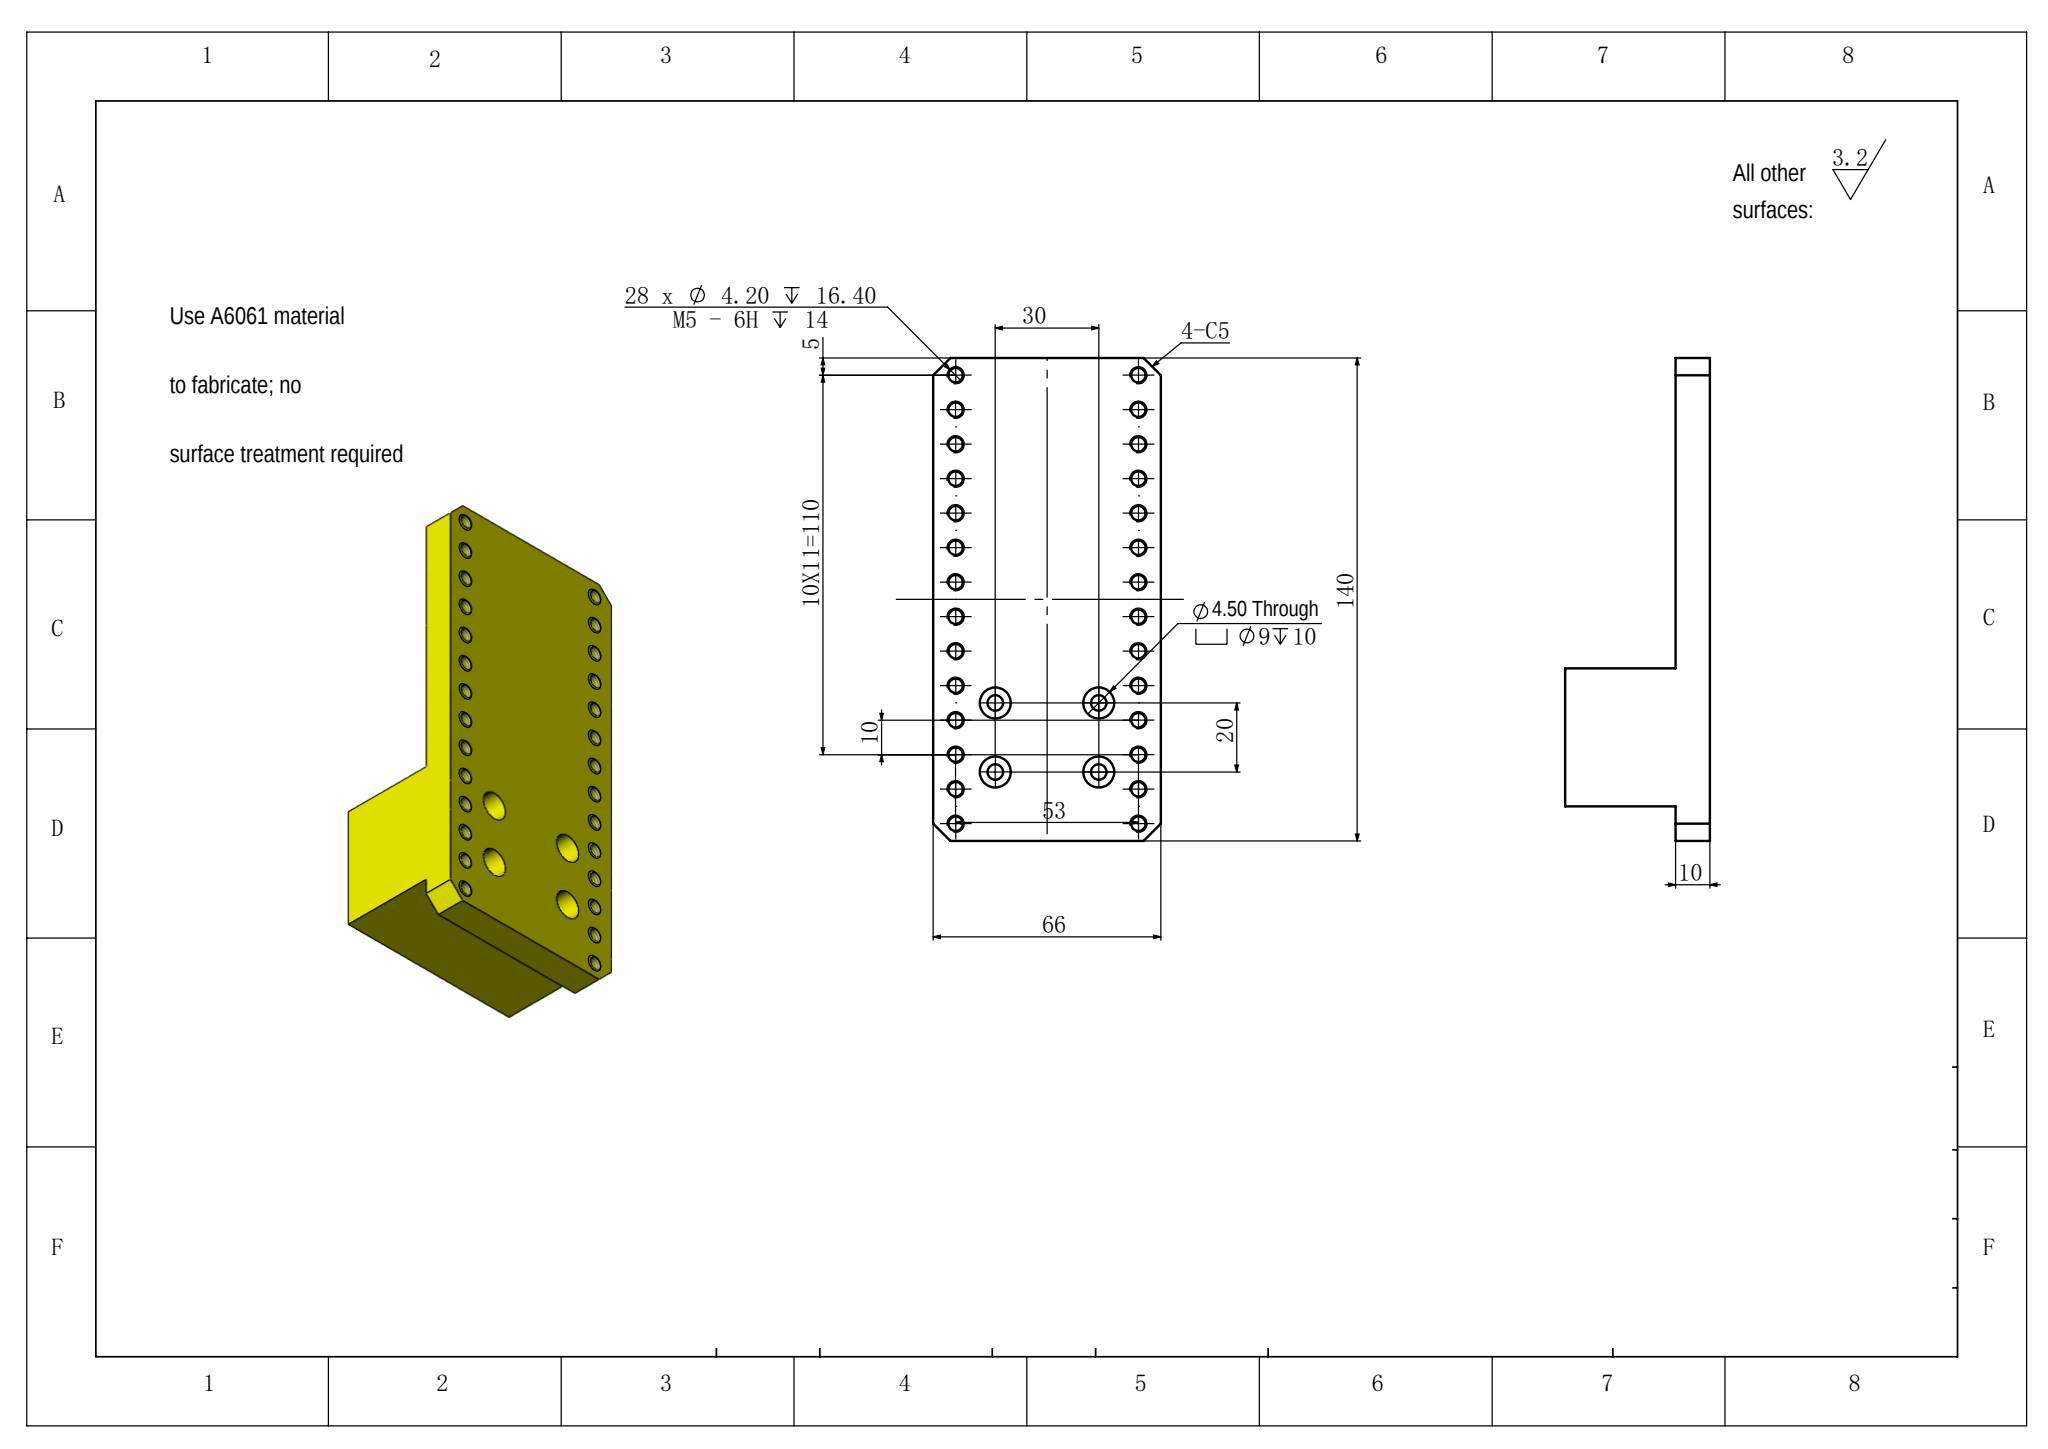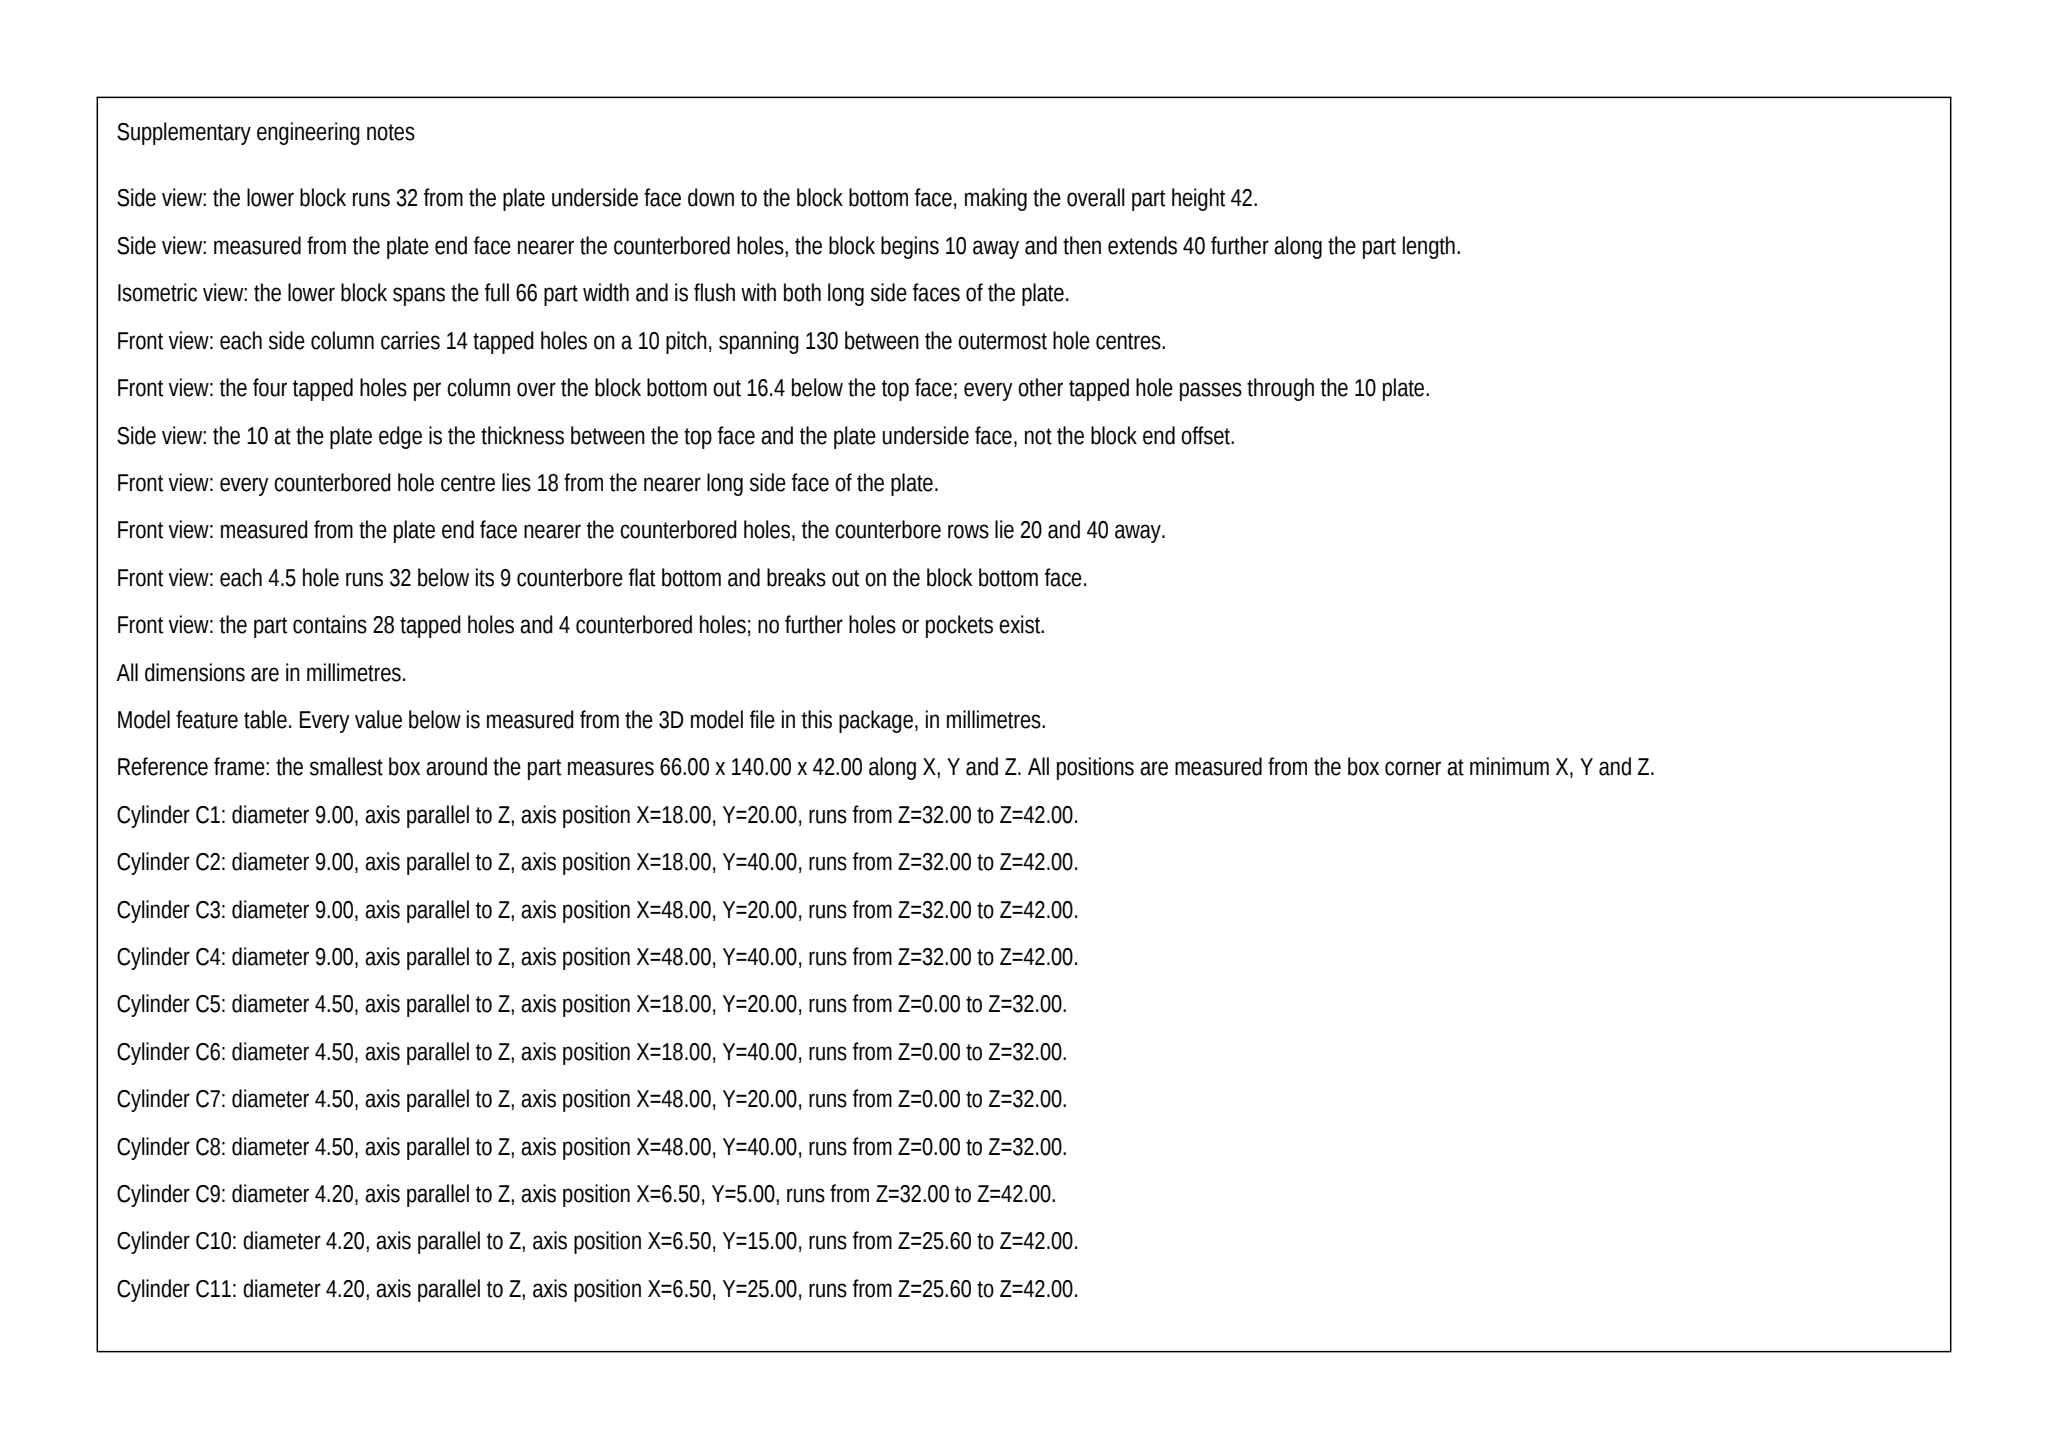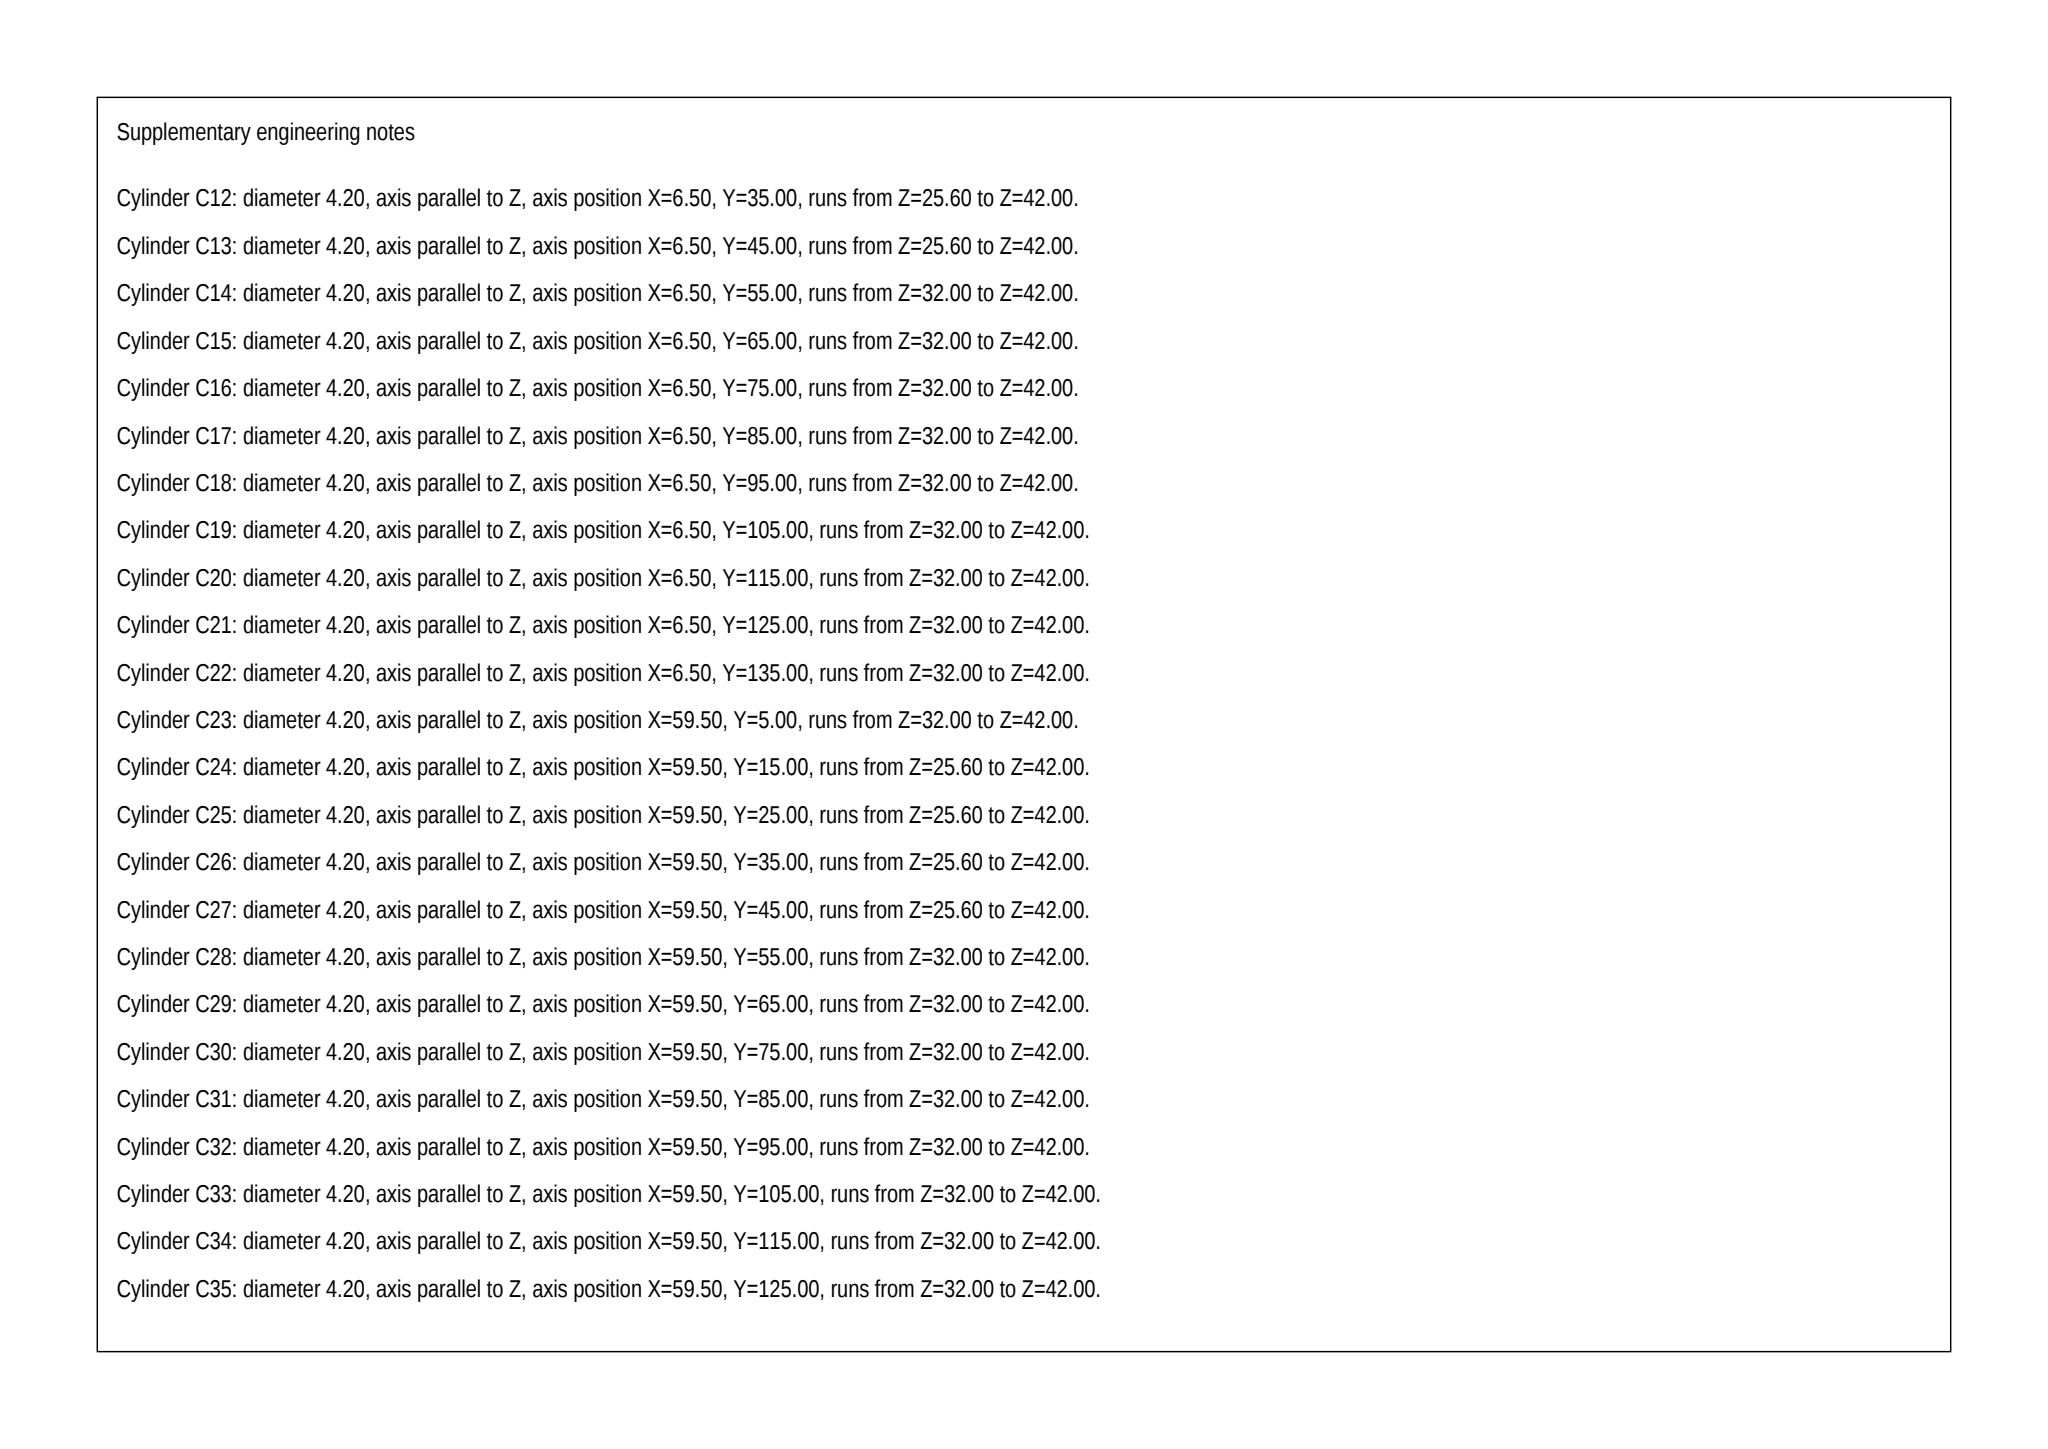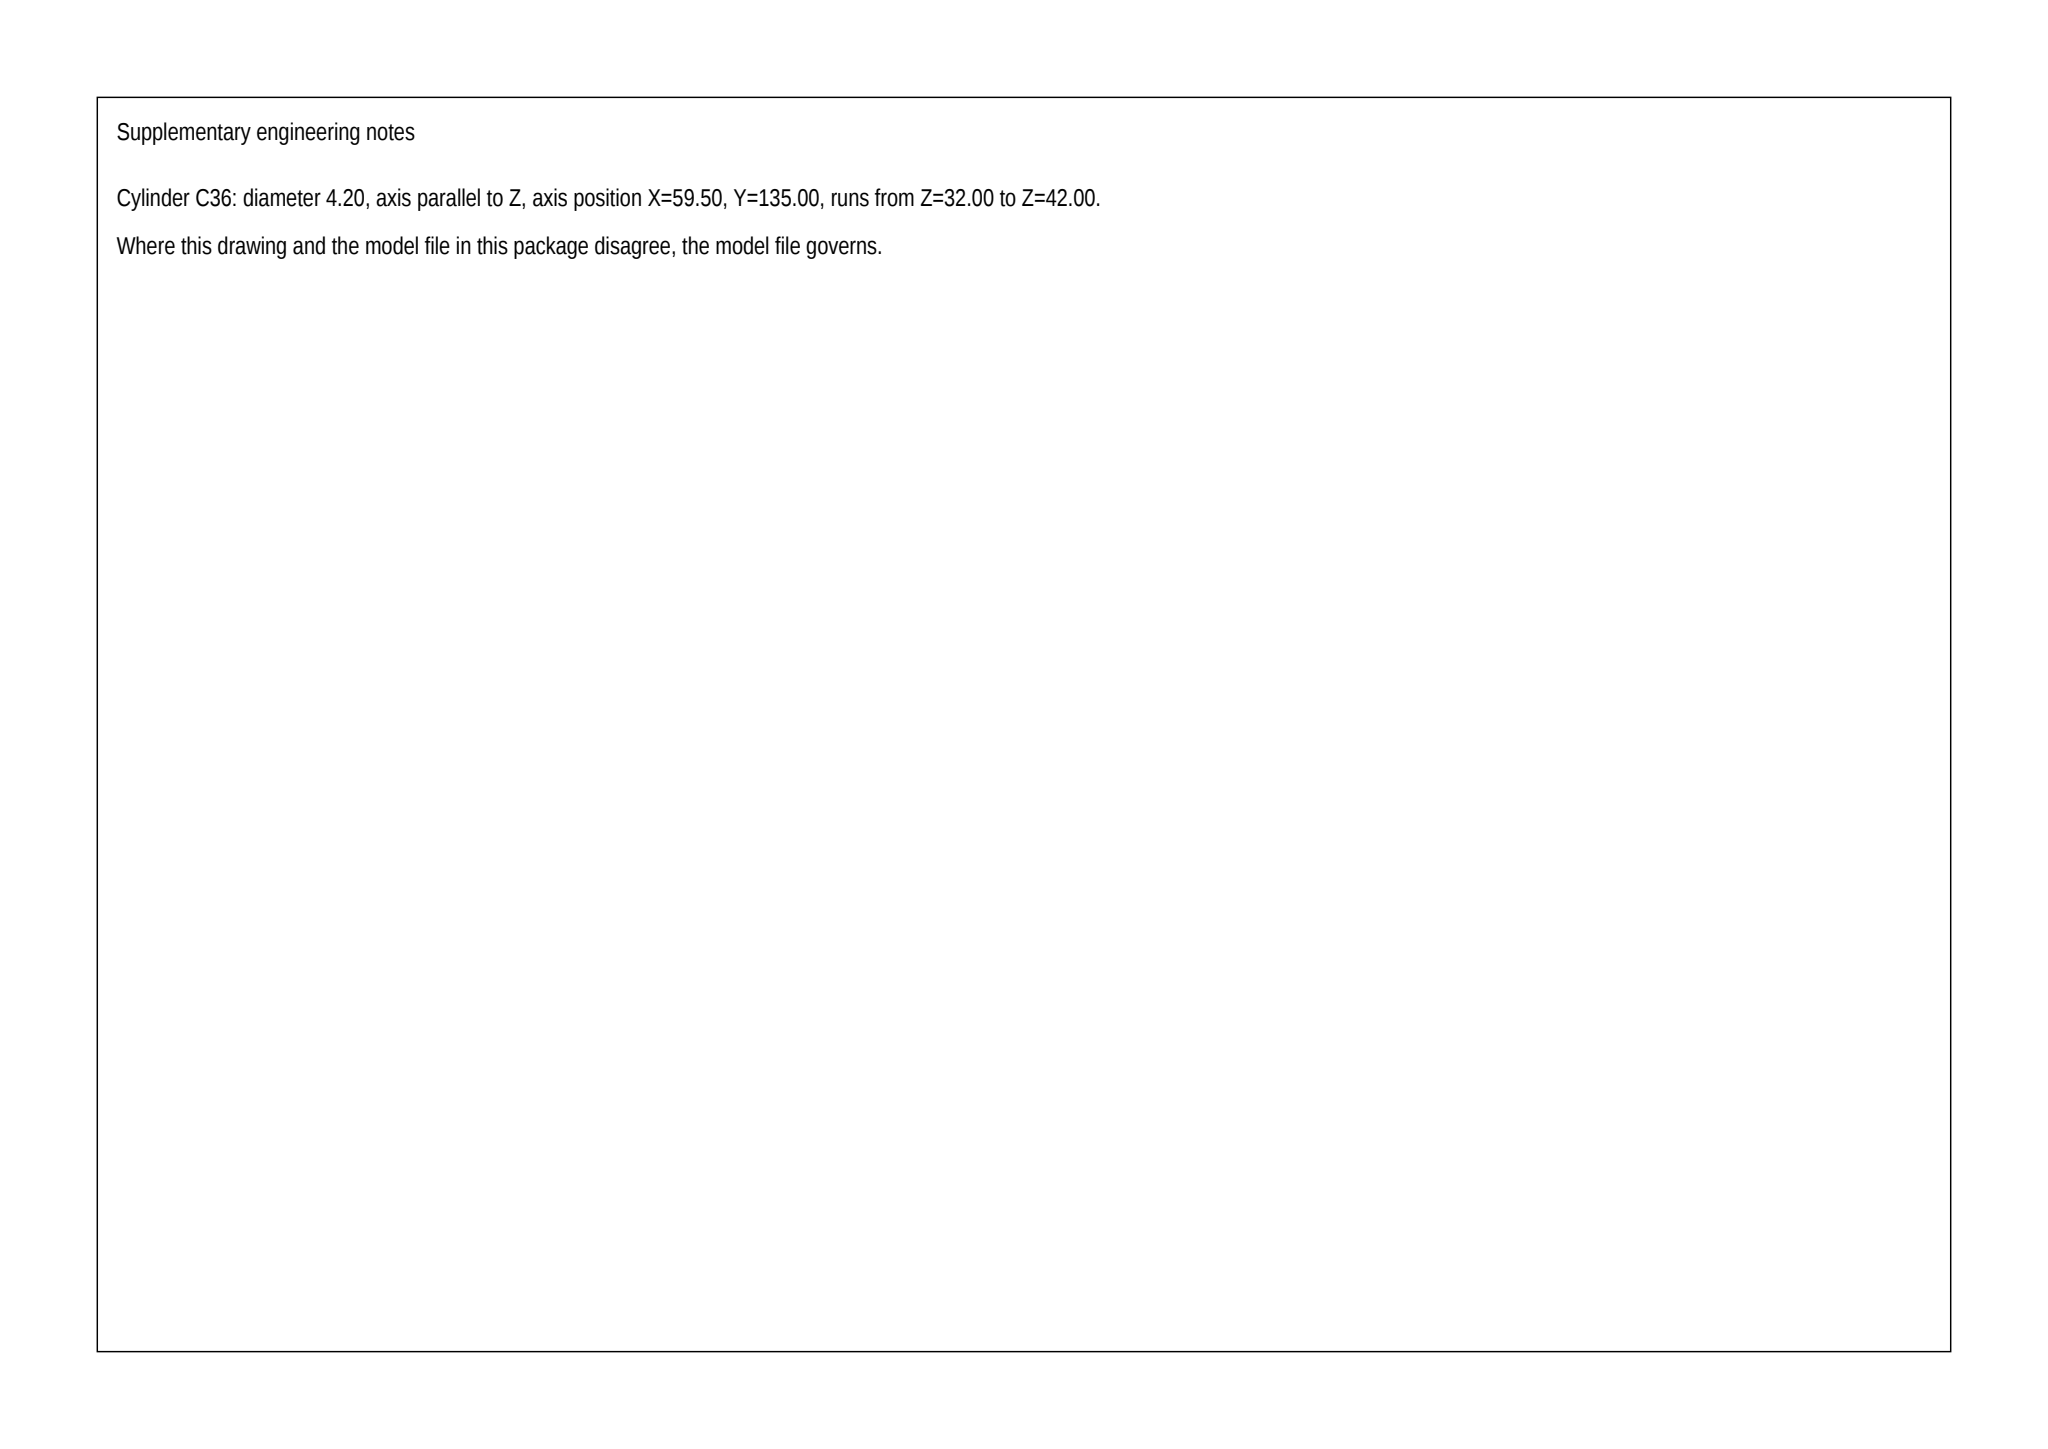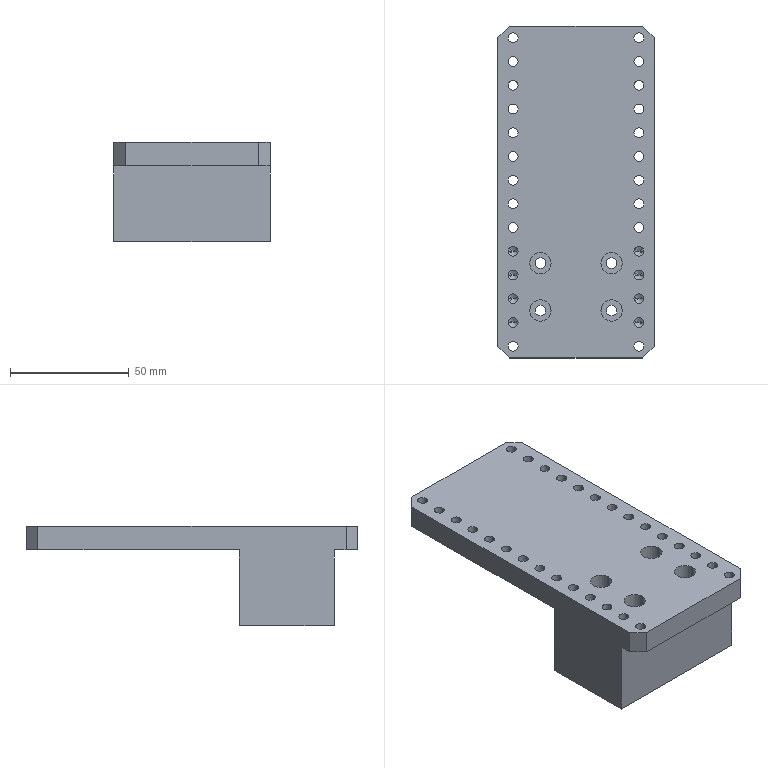Part | SolidWorks | mm | 1 solid | 106 faces | box 66 x 140 x 42 mm | volume 167164 mm3 | cylinder 72 | plane 18 | cone 16 | commonest cylinder face diameters 4.2 x56 9 x8 4.5 x8
Drawing notes:
SIDE VIEW: OVERALL DEPTH 42 | from the solid: bbox_xyz z = 42.0
BOSS PROJECTS 32 FROM PLATE BACK FACE | from the solid: z planes at 0.0 and 32.0; plate 32.0-42.0
BOSS 40 LG IN 140 DIR | from the solid: y planes at 10.0 and 50.0
BOSS STARTS 10 FROM BOTTOM EDGE | from the solid: y plane at 10.0 vs y=0 bottom edge
4X CBORED HOLES: LOWER ROW 20 FROM BOTTOM EDGE | from the solid: Ø4.5/Ø9 holes at y=20.0 and y=40.0
Ø4.50 DP 32 THRU BOSS, CBORE Ø9 DP 10 FROM FRONT FACE | from the solid: Ø4.5 L=32 from z=0; Ø9 L=10 in plate
20X M5-6H THRU (Ø4.20 THRU 10 PLATE); 8X IN BOSS Ø4.20 DP 16.40 M5 DP 14 | from the solid: Ø4.2 L=10 at y=5,55..135; Ø4.2 L=16.4 at y=15,25,35,45
BOSS FULL 66 WIDE ACROSS X (FLUSH BOTH SIDES), 10 THK | from the solid: bbox X=66; boss planes z=32 & z=42 span x=0..66, no x-offset faces
EA COL: 14 HOLES, 5 FROM BOTTOM EDGE, 13X10=130, 5 TO TOP | from the solid: 4.2 dia holes at y=5,15,...,135 (14 per col), bbox Y=140
8X M5-6H DP 14 (Ø4.20 DP 16.40) AT Y=15,25,35,45 EA COL; OTHER 20 DP 10 | from the solid: len 16.4 only at y=15,25,35,45 for x=6.5 & 59.5; remaining 4.2 holes len 10
build123d program:
from build123d import *

# Parameters (mm, degrees)
SKETCH1_W                  = 66
SKETCH1_H                  = 140
BOSS_EXTRUDE1_DEPTH        = 42
M5_TAPPED_HOLE1_AT_2_COUNT = 2
M5_TAPPED_HOLE1_AT_2_PITCH = 53
LPATTERN1_COUNT            = 14
LPATTERN1_PITCH            = 10
SKETCH4_R                  = 2.25
CUT_EXTRUDE1_DEPTH         = 89.051
CHAMFER1_SIZE              = 5
SKETCH5_R                  = 4.5
CUT_EXTRUDE2_DEPTH         = 10
SKETCH7_W                  = 47.361
SKETCH7_H                  = 127.61
SKETCH7_W_2                = 37.143
SKETCH7_H_2                = 85.293
CUT_EXTRUDE3_DEPTH         = 105.976


with BuildPart() as part:
    # Sketch1 → Boss-Extrude1 (new body)
    with BuildSketch(Plane.XY):
        Rectangle(SKETCH1_W, SKETCH1_H)
    extrude(amount=BOSS_EXTRUDE1_DEPTH)

    # Sketch3 → M5 Tapped Hole1 (revolve, cut)
    with BuildSketch(Plane(origin=(-26.5, 65, 42), x_dir=(0, -1, 0), z_dir=(1, 0, 0))):
        Polygon((0, 0), (0, 17.662), (2.1, 16.4), (2.1, 0), align=None)
    m5_tapped_hole1 = revolve(axis=Axis((-26.5, 65, 48.35), (0, 0, -1)), mode=Mode.SUBTRACT)

    # M5 Tapped Hole1 at 2: M5 Tapped Hole1 ×2
    with Locations(*[(i * M5_TAPPED_HOLE1_AT_2_PITCH, 0, 0) for i in range(1, M5_TAPPED_HOLE1_AT_2_COUNT)]):
        add(m5_tapped_hole1, mode=Mode.SUBTRACT)

    # LPattern1: M5 Tapped Hole1 ×14
    with Locations(*[(0, -i * LPATTERN1_PITCH, 0) for i in range(1, LPATTERN1_COUNT)]):
        add(m5_tapped_hole1, mode=Mode.SUBTRACT)

    # LPattern1 copy 1 sketch → LPattern1 copy 1 (revolve, cut)
    with BuildSketch(Plane(origin=(26.5, 55, 42), x_dir=(0, -1, 0), z_dir=(1, 0, 0))):
        Polygon((0, 0), (0, 17.662), (2.1, 16.4), (2.1, 0), align=None)
    revolve(axis=Axis((26.5, 55, 48.35), (0, 0, -1)), mode=Mode.SUBTRACT)

    # LPattern1 copy 2 sketch → LPattern1 copy 2 (revolve, cut)
    with BuildSketch(Plane(origin=(26.5, 45, 42), x_dir=(0, -1, 0), z_dir=(1, 0, 0))):
        Polygon((0, 0), (0, 17.662), (2.1, 16.4), (2.1, 0), align=None)
    revolve(axis=Axis((26.5, 45, 48.35), (0, 0, -1)), mode=Mode.SUBTRACT)

    # LPattern1 copy 3 sketch → LPattern1 copy 3 (revolve, cut)
    with BuildSketch(Plane(origin=(26.5, 35, 42), x_dir=(0, -1, 0), z_dir=(1, 0, 0))):
        Polygon((0, 0), (0, 17.662), (2.1, 16.4), (2.1, 0), align=None)
    revolve(axis=Axis((26.5, 35, 48.35), (0, 0, -1)), mode=Mode.SUBTRACT)

    # LPattern1 copy 4 sketch → LPattern1 copy 4 (revolve, cut)
    with BuildSketch(Plane(origin=(26.5, 25, 42), x_dir=(0, -1, 0), z_dir=(1, 0, 0))):
        Polygon((0, 0), (0, 17.662), (2.1, 16.4), (2.1, 0), align=None)
    revolve(axis=Axis((26.5, 25, 48.35), (0, 0, -1)), mode=Mode.SUBTRACT)

    # LPattern1 copy 5 sketch → LPattern1 copy 5 (revolve, cut)
    with BuildSketch(Plane(origin=(26.5, 15, 42), x_dir=(0, -1, 0), z_dir=(1, 0, 0))):
        Polygon((0, 0), (0, 17.662), (2.1, 16.4), (2.1, 0), align=None)
    revolve(axis=Axis((26.5, 15, 48.35), (0, 0, -1)), mode=Mode.SUBTRACT)

    # LPattern1 copy 6 sketch → LPattern1 copy 6 (revolve, cut)
    with BuildSketch(Plane(origin=(26.5, 5, 42), x_dir=(0, -1, 0), z_dir=(1, 0, 0))):
        Polygon((0, 0), (0, 17.662), (2.1, 16.4), (2.1, 0), align=None)
    revolve(axis=Axis((26.5, 5, 48.35), (0, 0, -1)), mode=Mode.SUBTRACT)

    # LPattern1 copy 7 sketch → LPattern1 copy 7 (revolve, cut)
    with BuildSketch(Plane(origin=(26.5, -5, 42), x_dir=(0, -1, 0), z_dir=(1, 0, 0))):
        Polygon((0, 0), (0, 17.662), (2.1, 16.4), (2.1, 0), align=None)
    revolve(axis=Axis((26.5, -5, 48.35), (0, 0, -1)), mode=Mode.SUBTRACT)

    # LPattern1 copy 8 sketch → LPattern1 copy 8 (revolve, cut)
    with BuildSketch(Plane(origin=(26.5, -15, 42), x_dir=(0, -1, 0), z_dir=(1, 0, 0))):
        Polygon((0, 0), (0, 17.662), (2.1, 16.4), (2.1, 0), align=None)
    revolve(axis=Axis((26.5, -15, 48.35), (0, 0, -1)), mode=Mode.SUBTRACT)

    # LPattern1 copy 9 sketch → LPattern1 copy 9 (revolve, cut)
    with BuildSketch(Plane(origin=(26.5, -25, 42), x_dir=(0, -1, 0), z_dir=(1, 0, 0))):
        Polygon((0, 0), (0, 17.662), (2.1, 16.4), (2.1, 0), align=None)
    revolve(axis=Axis((26.5, -25, 48.35), (0, 0, -1)), mode=Mode.SUBTRACT)

    # LPattern1 copy 10 sketch → LPattern1 copy 10 (revolve, cut)
    with BuildSketch(Plane(origin=(26.5, -35, 42), x_dir=(0, -1, 0), z_dir=(1, 0, 0))):
        Polygon((0, 0), (0, 17.662), (2.1, 16.4), (2.1, 0), align=None)
    revolve(axis=Axis((26.5, -35, 48.35), (0, 0, -1)), mode=Mode.SUBTRACT)

    # LPattern1 copy 11 sketch → LPattern1 copy 11 (revolve, cut)
    with BuildSketch(Plane(origin=(26.5, -45, 42), x_dir=(0, -1, 0), z_dir=(1, 0, 0))):
        Polygon((0, 0), (0, 17.662), (2.1, 16.4), (2.1, 0), align=None)
    revolve(axis=Axis((26.5, -45, 48.35), (0, 0, -1)), mode=Mode.SUBTRACT)

    # LPattern1 copy 12 sketch → LPattern1 copy 12 (revolve, cut)
    with BuildSketch(Plane(origin=(26.5, -55, 42), x_dir=(0, -1, 0), z_dir=(1, 0, 0))):
        Polygon((0, 0), (0, 17.662), (2.1, 16.4), (2.1, 0), align=None)
    revolve(axis=Axis((26.5, -55, 48.35), (0, 0, -1)), mode=Mode.SUBTRACT)

    # LPattern1 copy 13 sketch → LPattern1 copy 13 (revolve, cut)
    with BuildSketch(Plane(origin=(26.5, -65, 42), x_dir=(0, -1, 0), z_dir=(1, 0, 0))):
        Polygon((0, 0), (0, 17.662), (2.1, 16.4), (2.1, 0), align=None)
    revolve(axis=Axis((26.5, -65, 48.35), (0, 0, -1)), mode=Mode.SUBTRACT)

    # Sketch4 → Cut-Extrude1 (cut, through all)
    with BuildSketch(Plane.XY.offset(42)):
        with Locations((-15, -30)):
            Circle(SKETCH4_R)
        with Locations((15, -30)):
            Circle(SKETCH4_R)
        with Locations((-15, -50)):
            Circle(SKETCH4_R)
        with Locations((15, -50)):
            Circle(SKETCH4_R)
    extrude(amount=-CUT_EXTRUDE1_DEPTH, mode=Mode.SUBTRACT)

    # Chamfer1
    chamfer1_edges = [part.edges().sort_by_distance(p)[0] for p in [
        (33, -70, 21),
        (-33, -70, 21),
        (-33, 70, 21),
        (33, 70, 21),
    ]]
    chamfer(chamfer1_edges, length=CHAMFER1_SIZE)

    # Sketch5 → Cut-Extrude2 (cut)
    with BuildSketch(Plane.XY.offset(42)):
        with Locations((-15, -30)):
            Circle(SKETCH5_R)
        with Locations((-15, -50)):
            Circle(SKETCH5_R)
        with Locations((15, -30)):
            Circle(SKETCH5_R)
        with Locations((15, -50)):
            Circle(SKETCH5_R)
    extrude(amount=-CUT_EXTRUDE2_DEPTH, mode=Mode.SUBTRACT)

    # Sketch7 → Cut-Extrude3 (cut, through all)
    with BuildSketch(Plane.ZY.offset(33)):
        with Locations((8.32, 43.805)):
            Rectangle(SKETCH7_W, SKETCH7_H)
        with Locations((13.429, -102.647)):
            Rectangle(SKETCH7_W_2, SKETCH7_H_2)
    extrude(amount=-CUT_EXTRUDE3_DEPTH, mode=Mode.SUBTRACT)


solid = part.part